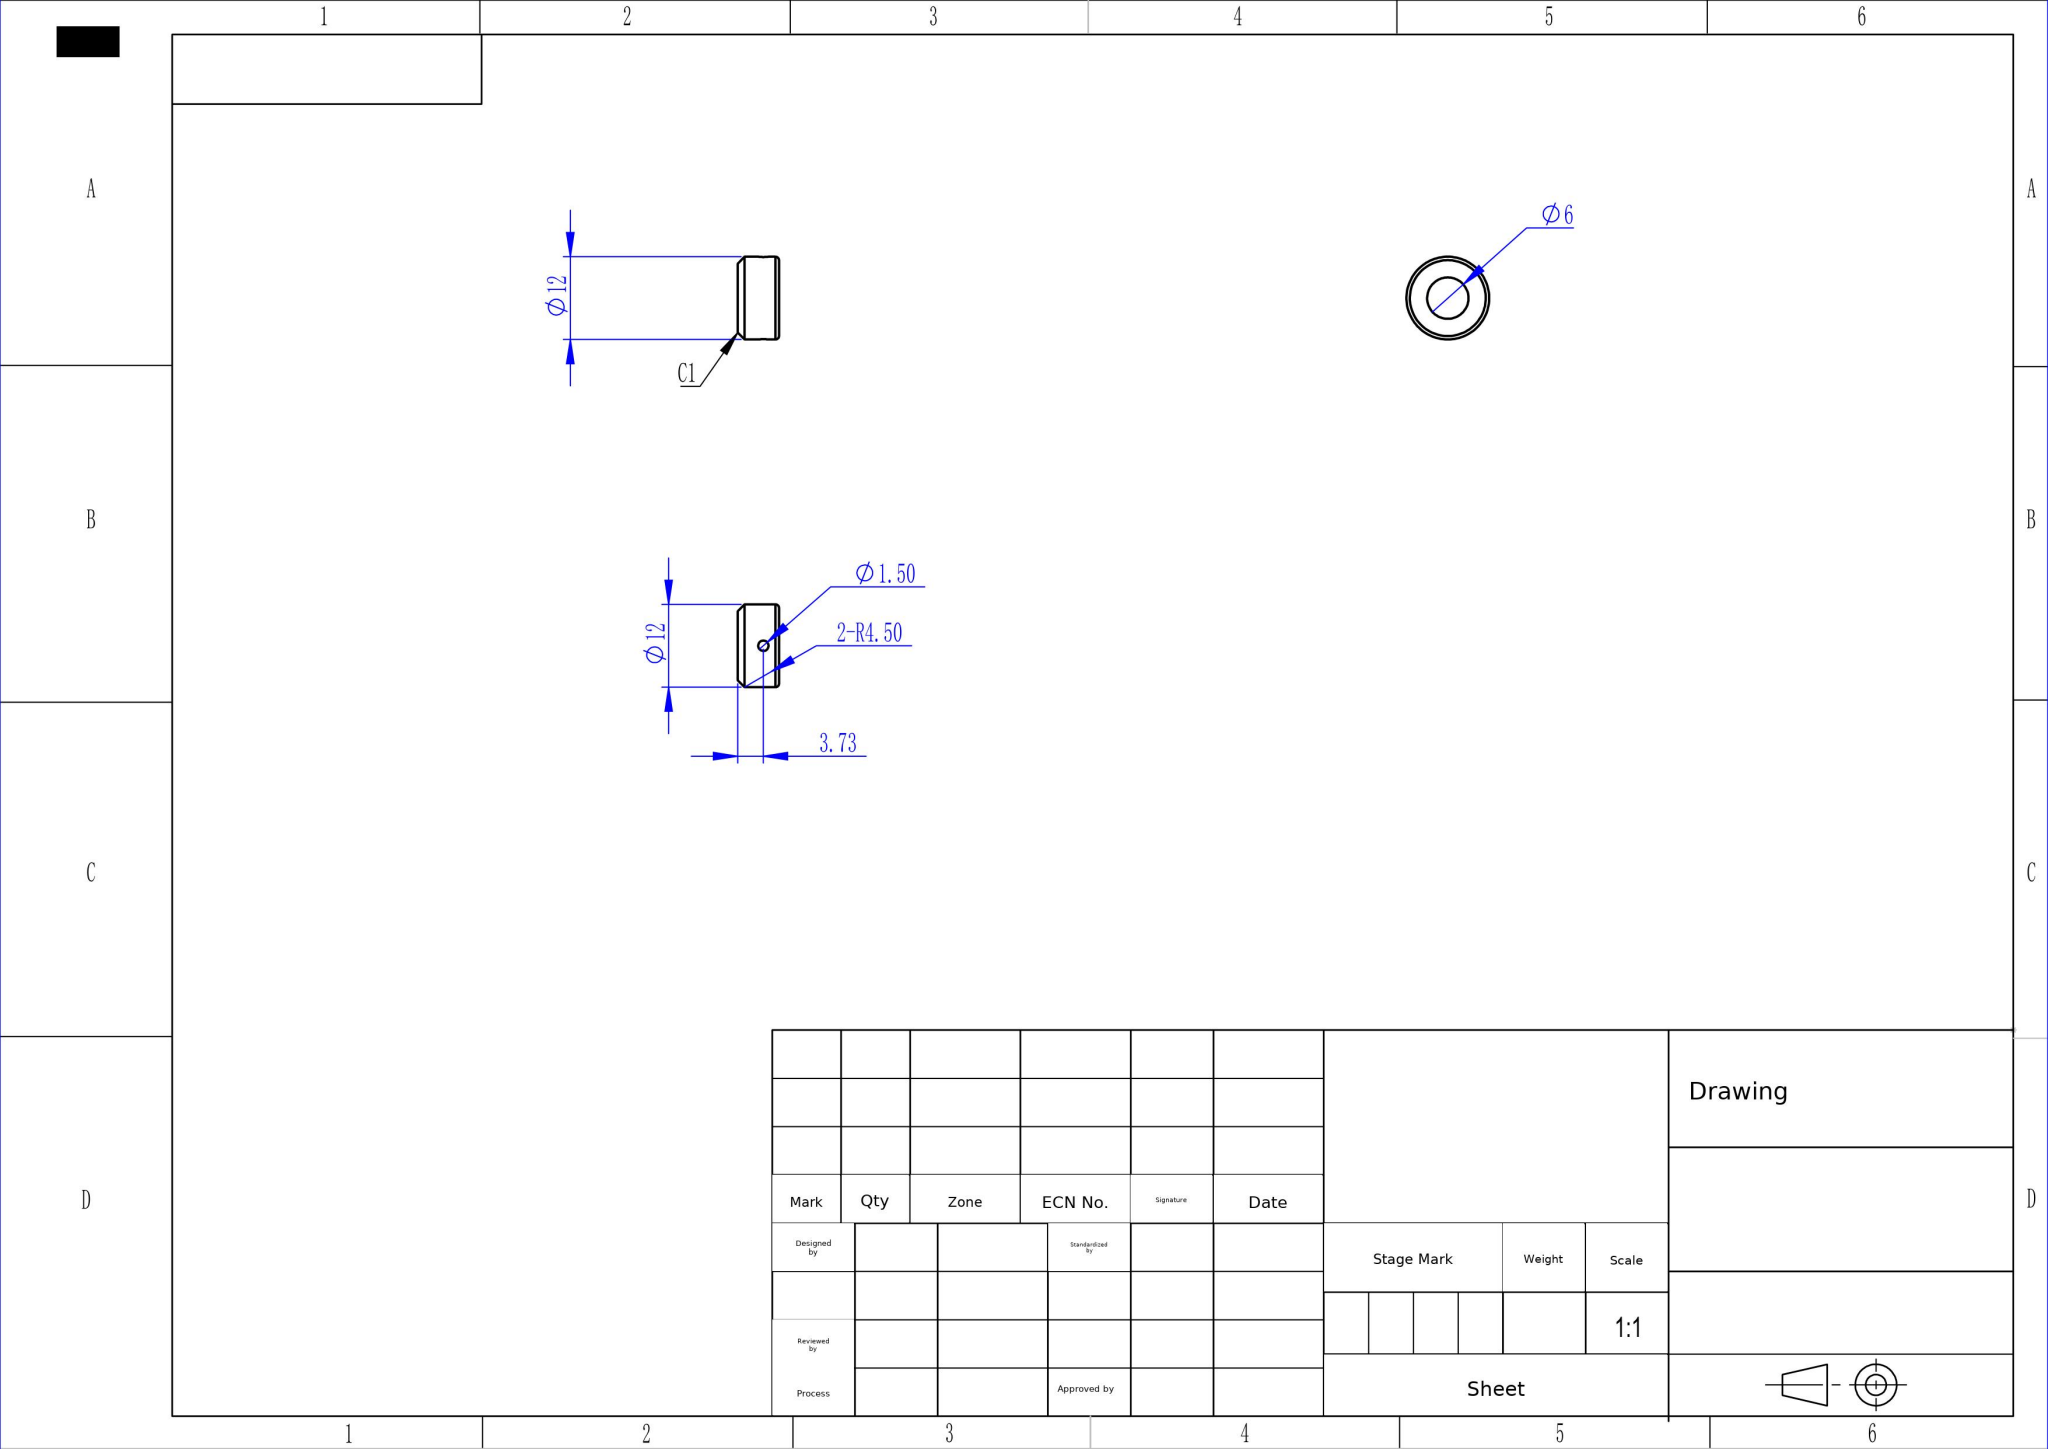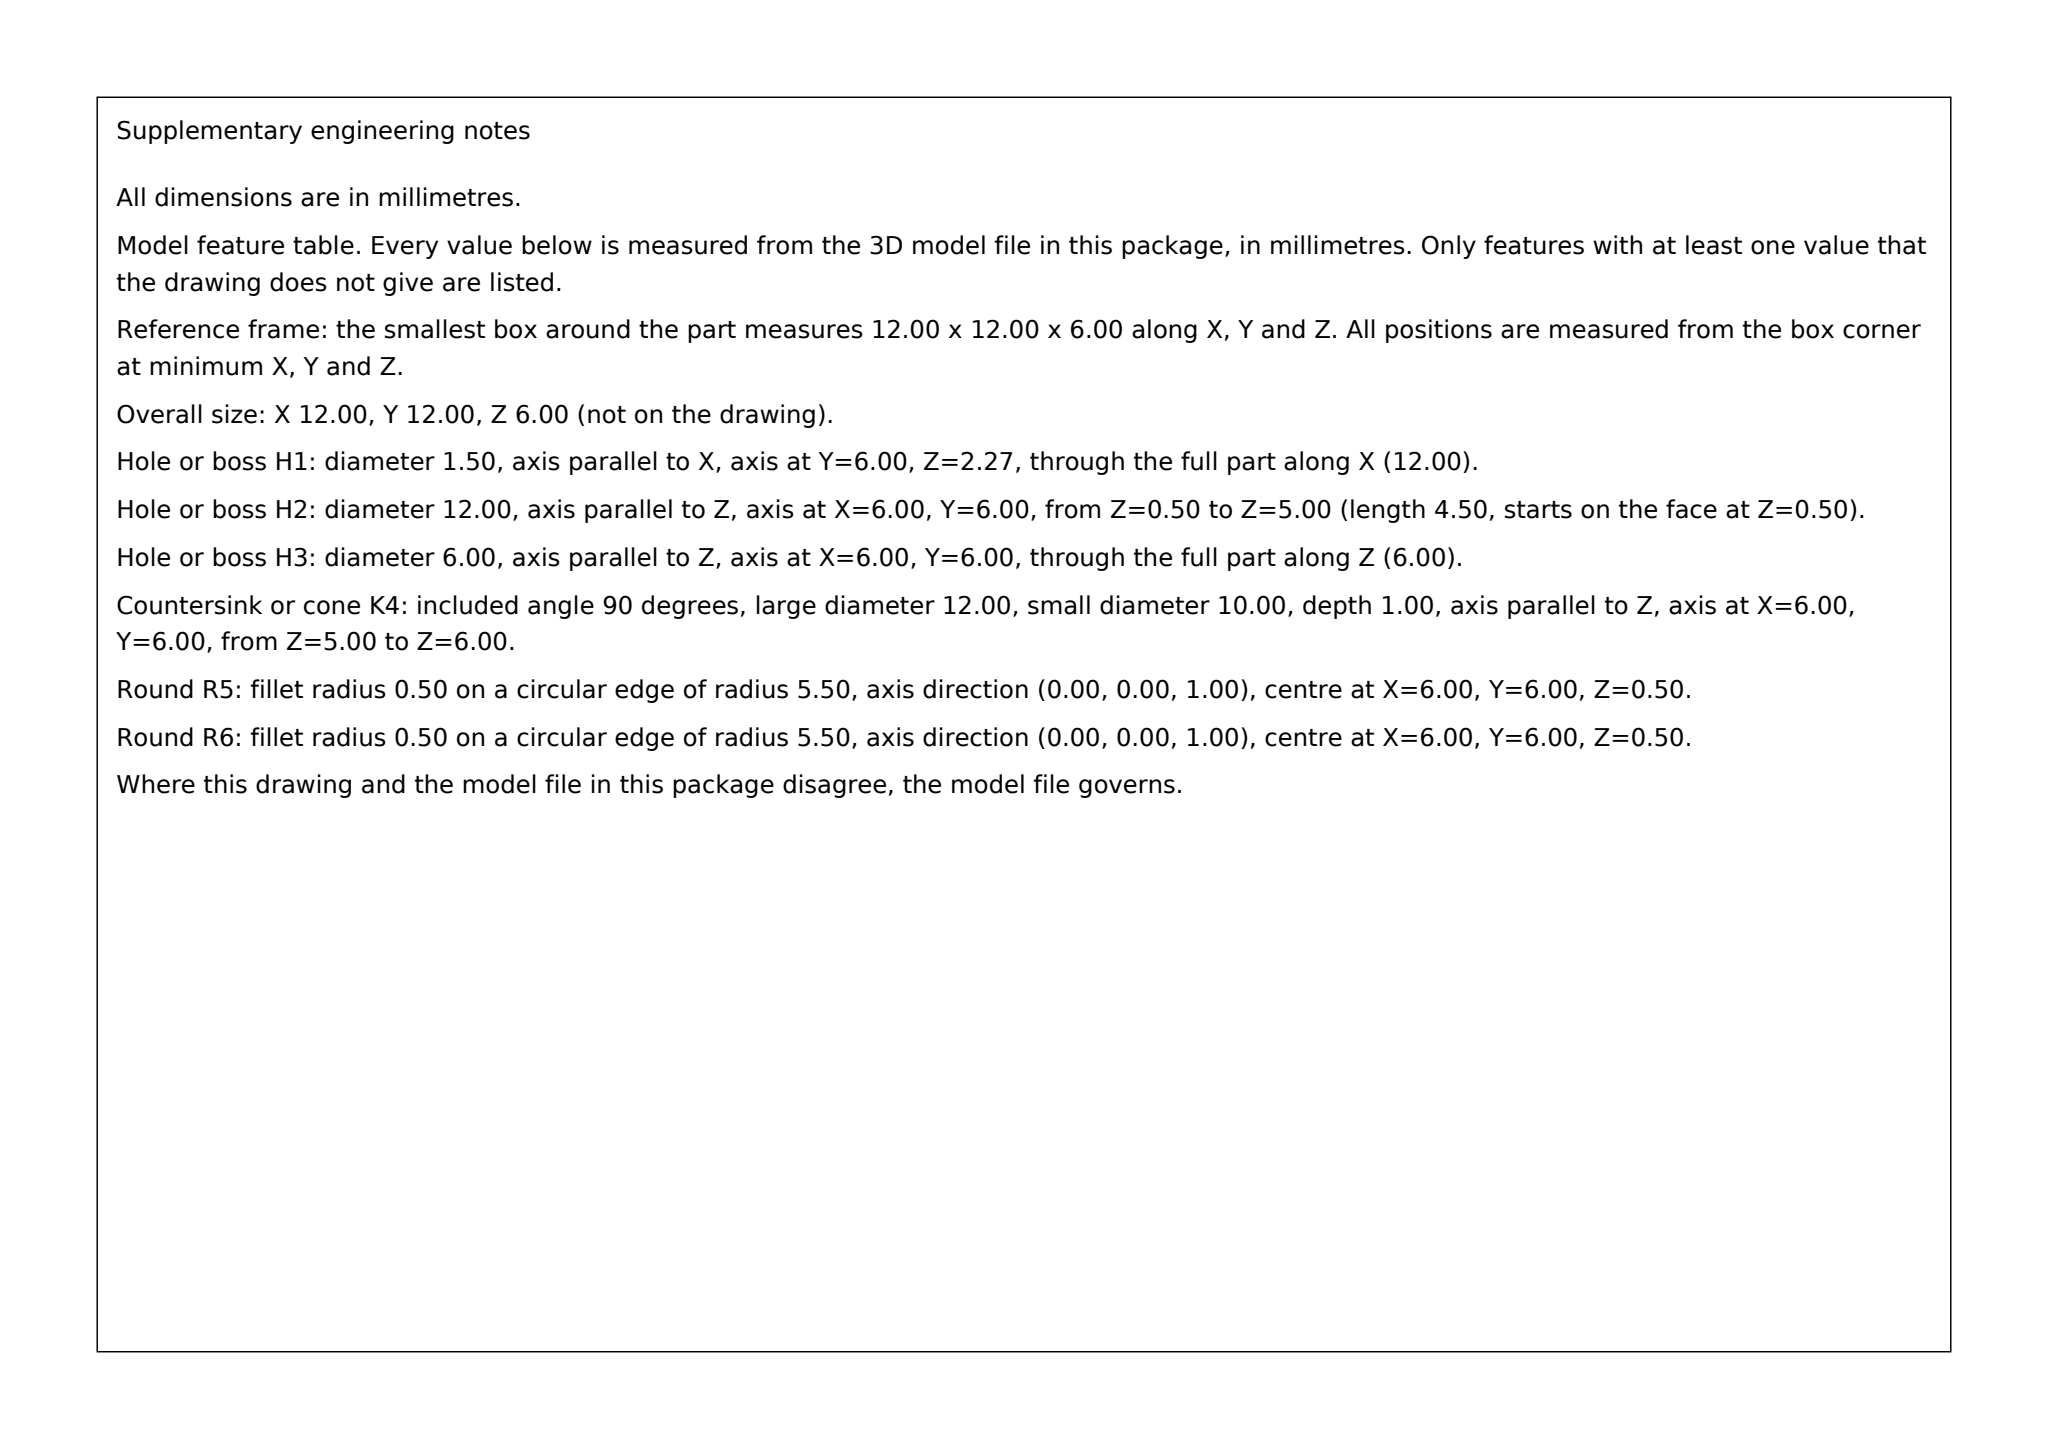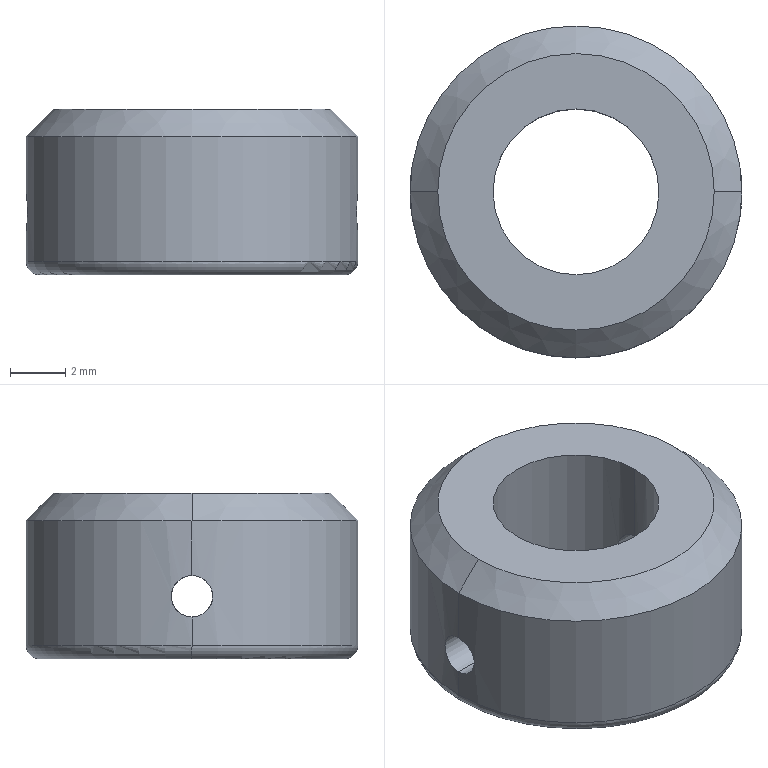Part | SolidWorks | mm | 1 solid | 14 faces | box 12 x 12 x 6 mm | volume 479 mm3 | cylinder 8 | cone 2 | torus 2 | plane 2 | commonest cylinder face diameters 1.5 x4 6 x2 12 x2
build123d program:
from build123d import *

# Parameters (mm, degrees)
SKETCH1_R               = 6
SKETCH1_R_2             = 3
BOSS_EXTRUDE1_DEPTH     = 6
FILLET1_R               = 0.5
CHAMFER1_SIZE           = 1
CUT_EXTRUDE1_DEPTH      = 11.392
CUT_EXTRUDE1_DEPTH_BACK = 11.392
SKETCH2_R               = 0.75


with BuildPart() as part:
    # Sketch1 → Boss-Extrude1 (new body)
    with BuildSketch(Plane.XY):
        Circle(SKETCH1_R)
        Circle(SKETCH1_R_2, mode=Mode.SUBTRACT)
    extrude(amount=BOSS_EXTRUDE1_DEPTH)

    # Fillet1
    fillet1_edges = [part.edges().sort_by_distance(p)[0] for p in [
        (-6, 0, 0),
    ]]
    fillet(fillet1_edges, radius=FILLET1_R)

    # Chamfer1
    chamfer1_edges = [part.edges().sort_by_distance(p)[0] for p in [
        (-6, 0, 6),
    ]]
    chamfer(chamfer1_edges, length=CHAMFER1_SIZE)

    # Sketch2 → Cut-Extrude1 (cut, two sides: drawn at the far end of the back side and taken through both)
    with BuildSketch(Plane(origin=(0, 0, 0), x_dir=(0, 0, -1), z_dir=(1, 0, 0)).offset(-CUT_EXTRUDE1_DEPTH_BACK)):
        with Locations((-2.267, 0)):
            Circle(SKETCH2_R)
    extrude(amount=CUT_EXTRUDE1_DEPTH + CUT_EXTRUDE1_DEPTH_BACK, mode=Mode.SUBTRACT)


solid = part.part
STEP:
#1=CARTESIAN_POINT('',(-6.,0.,3.017));
#2=VERTEX_POINT('',#1);
#3=CARTESIAN_POINT('',(-6.,0.,1.517));
#4=VERTEX_POINT('',#3);
#5=CARTESIAN_POINT('',(-6.,0.,3.017));
#6=CARTESIAN_POINT('',(-6.,-0.1958,3.017));
#7=CARTESIAN_POINT('',(-5.989,-0.3916,2.936));
#8=CARTESIAN_POINT('',(-5.97,-0.5992,2.729));
#9=CARTESIAN_POINT('',(-5.964,-0.6549,2.646));
#10=CARTESIAN_POINT('',(-5.956,-0.7303,2.464));
#11=CARTESIAN_POINT('',(-5.953,-0.7499,2.367));
#12=CARTESIAN_POINT('',(-5.953,-0.7501,2.169));
#13=CARTESIAN_POINT('',(-5.955,-0.7306,2.071));
#14=CARTESIAN_POINT('',(-5.964,-0.6554,1.89));
#15=CARTESIAN_POINT('',(-5.97,-0.5997,1.806));
#16=CARTESIAN_POINT('',(-5.989,-0.3926,1.599));
#17=CARTESIAN_POINT('',(-6.,-0.1984,1.517));
#18=CARTESIAN_POINT('',(-6.,0.,1.517));
#19=B_SPLINE_CURVE_WITH_KNOTS('',3,(#5,#6,#7,#8,#9,#10,#11,#12,#13,#14,#15,#16,#17,#18),.UNSPECIFIED.,.F.,.F.,(4,2,2,2,2,2,4),(0.002347,0.002934,0.003227,0.00352,0.003814,0.004107,0.004694),.UNSPECIFIED.);
#20=EDGE_CURVE('',#2,#4,#19,.T.);
#21=ORIENTED_EDGE('',*,*,#20,.F.);
#22=CARTESIAN_POINT('',(-3.,0.,3.017));
#23=VERTEX_POINT('',#22);
#24=CARTESIAN_POINT('',(-6.,0.,3.017));
#25=DIRECTION('',(1.,0.,0.));
#26=VECTOR('',#25,1000.);
#27=LINE('',#24,#26);
#28=EDGE_CURVE('',#2,#23,#27,.T.);
#29=ORIENTED_EDGE('',*,*,#28,.T.);
#30=CARTESIAN_POINT('',(-3.,0.,1.517));
#31=VERTEX_POINT('',#30);
#32=CARTESIAN_POINT('',(-3.,0.,3.017));
#33=CARTESIAN_POINT('',(-3.,-0.09953,3.017));
#34=CARTESIAN_POINT('',(-2.995,-0.1972,2.998));
#35=CARTESIAN_POINT('',(-2.977,-0.3787,2.922));
#36=CARTESIAN_POINT('',(-2.965,-0.4616,2.866));
#37=CARTESIAN_POINT('',(-2.94,-0.5994,2.729));
#38=CARTESIAN_POINT('',(-2.928,-0.6552,2.645));
#39=CARTESIAN_POINT('',(-2.91,-0.7301,2.465));
#40=CARTESIAN_POINT('',(-2.905,-0.75,2.366));
#41=CARTESIAN_POINT('',(-2.905,-0.75,2.169));
#42=CARTESIAN_POINT('',(-2.91,-0.7305,2.071));
#43=CARTESIAN_POINT('',(-2.928,-0.6549,1.889));
#44=CARTESIAN_POINT('',(-2.94,-0.5997,1.806));
#45=CARTESIAN_POINT('',(-2.965,-0.4607,1.667));
#46=CARTESIAN_POINT('',(-2.977,-0.3781,1.612));
#47=CARTESIAN_POINT('',(-2.995,-0.197,1.537));
#48=CARTESIAN_POINT('',(-3.,-0.09813,1.517));
#49=CARTESIAN_POINT('',(-3.,0.,1.517));
#50=B_SPLINE_CURVE_WITH_KNOTS('',3,(#32,#33,#34,#35,#36,#37,#38,#39,#40,#41,#42,#43,#44,#45,#46,#47,#48,#49),.UNSPECIFIED.,.F.,.F.,(4,2,2,2,2,2,2,2,4),(0.,0.0002943,0.0005886,0.0008828,0.001177,0.001471,0.001766,0.00206,0.002354),.UNSPECIFIED.);
#51=EDGE_CURVE('',#23,#31,#50,.T.);
#52=ORIENTED_EDGE('',*,*,#51,.T.);
#53=CARTESIAN_POINT('',(-6.,0.,1.517));
#54=DIRECTION('',(1.,0.,0.));
#55=VECTOR('',#54,1000.);
#56=LINE('',#53,#55);
#57=EDGE_CURVE('',#4,#31,#56,.T.);
#58=ORIENTED_EDGE('',*,*,#57,.F.);
#59=EDGE_LOOP('',(#21,#29,#52,#58));
#60=FACE_OUTER_BOUND('',#59,.T.);
#61=CARTESIAN_POINT('',(-6.,0.,2.267));
#62=DIRECTION('',(1.,0.,0.));
#63=DIRECTION('',(0.,0.,-1.));
#64=AXIS2_PLACEMENT_3D('',#61,#62,#63);
#65=CYLINDRICAL_SURFACE('',#64,0.75);
#66=ADVANCED_FACE('',(#60),#65,.F.);
#67=CARTESIAN_POINT('',(3.,-0.,1.517));
#68=VERTEX_POINT('',#67);
#69=CARTESIAN_POINT('',(3.,0.,3.017));
#70=VERTEX_POINT('',#69);
#71=CARTESIAN_POINT('',(3.,-0.,1.517));
#72=CARTESIAN_POINT('',(3.,-0.09953,1.517));
#73=CARTESIAN_POINT('',(2.995,-0.1972,1.537));
#74=CARTESIAN_POINT('',(2.977,-0.3787,1.612));
#75=CARTESIAN_POINT('',(2.965,-0.4616,1.668));
#76=CARTESIAN_POINT('',(2.94,-0.5994,1.806));
#77=CARTESIAN_POINT('',(2.928,-0.6552,1.889));
#78=CARTESIAN_POINT('',(2.91,-0.7301,2.07));
#79=CARTESIAN_POINT('',(2.905,-0.75,2.169));
#80=CARTESIAN_POINT('',(2.905,-0.75,2.365));
#81=CARTESIAN_POINT('',(2.91,-0.7305,2.464));
#82=CARTESIAN_POINT('',(2.928,-0.6549,2.646));
#83=CARTESIAN_POINT('',(2.94,-0.5997,2.728));
#84=CARTESIAN_POINT('',(2.965,-0.4607,2.867));
#85=CARTESIAN_POINT('',(2.977,-0.3781,2.922));
#86=CARTESIAN_POINT('',(2.995,-0.197,2.998));
#87=CARTESIAN_POINT('',(3.,-0.09813,3.017));
#88=CARTESIAN_POINT('',(3.,0.,3.017));
#89=B_SPLINE_CURVE_WITH_KNOTS('',3,(#71,#72,#73,#74,#75,#76,#77,#78,#79,#80,#81,#82,#83,#84,#85,#86,#87,#88),.UNSPECIFIED.,.F.,.F.,(4,2,2,2,2,2,2,2,4),(0.,0.0002943,0.0005886,0.0008828,0.001177,0.001471,0.001766,0.00206,0.002354),.UNSPECIFIED.);
#90=EDGE_CURVE('',#68,#70,#89,.T.);
#91=ORIENTED_EDGE('',*,*,#90,.T.);
#92=CARTESIAN_POINT('',(6.,-0.,3.017));
#93=VERTEX_POINT('',#92);
#94=CARTESIAN_POINT('',(-6.,0.,3.017));
#95=DIRECTION('',(1.,0.,0.));
#96=VECTOR('',#95,1000.);
#97=LINE('',#94,#96);
#98=EDGE_CURVE('',#70,#93,#97,.T.);
#99=ORIENTED_EDGE('',*,*,#98,.T.);
#100=CARTESIAN_POINT('',(6.,0.,1.517));
#101=VERTEX_POINT('',#100);
#102=CARTESIAN_POINT('',(6.,0.,1.517));
#103=CARTESIAN_POINT('',(6.,-0.09921,1.517));
#104=CARTESIAN_POINT('',(5.997,-0.1966,1.537));
#105=CARTESIAN_POINT('',(5.989,-0.3782,1.612));
#106=CARTESIAN_POINT('',(5.983,-0.4613,1.668));
#107=CARTESIAN_POINT('',(5.964,-0.6687,1.875));
#108=CARTESIAN_POINT('',(5.953,-0.7499,2.071));
#109=CARTESIAN_POINT('',(5.953,-0.75,2.365));
#110=CARTESIAN_POINT('',(5.955,-0.7306,2.463));
#111=CARTESIAN_POINT('',(5.964,-0.6553,2.645));
#112=CARTESIAN_POINT('',(5.97,-0.6004,2.728));
#113=CARTESIAN_POINT('',(5.983,-0.4604,2.868));
#114=CARTESIAN_POINT('',(5.989,-0.3779,2.923));
#115=CARTESIAN_POINT('',(5.997,-0.1963,2.998));
#116=CARTESIAN_POINT('',(6.,-0.09795,3.017));
#117=CARTESIAN_POINT('',(6.,-0.,3.017));
#118=B_SPLINE_CURVE_WITH_KNOTS('',3,(#102,#103,#104,#105,#106,#107,#108,#109,#110,#111,#112,#113,#114,#115,#116,#117),.UNSPECIFIED.,.F.,.F.,(4,2,2,2,2,2,2,4),(0.,0.0002934,0.0005868,0.001174,0.001467,0.00176,0.002054,0.002347),.UNSPECIFIED.);
#119=EDGE_CURVE('',#101,#93,#118,.T.);
#120=ORIENTED_EDGE('',*,*,#119,.F.);
#121=CARTESIAN_POINT('',(-6.,0.,1.517));
#122=DIRECTION('',(1.,0.,0.));
#123=VECTOR('',#122,1000.);
#124=LINE('',#121,#123);
#125=EDGE_CURVE('',#68,#101,#124,.T.);
#126=ORIENTED_EDGE('',*,*,#125,.F.);
#127=EDGE_LOOP('',(#91,#99,#120,#126));
#128=FACE_OUTER_BOUND('',#127,.T.);
#129=CARTESIAN_POINT('',(-6.,0.,2.267));
#130=DIRECTION('',(1.,0.,0.));
#131=DIRECTION('',(0.,0.,-1.));
#132=AXIS2_PLACEMENT_3D('',#129,#130,#131);
#133=CYLINDRICAL_SURFACE('',#132,0.75);
#134=ADVANCED_FACE('',(#128),#133,.F.);
#135=CARTESIAN_POINT('',(5.,0.,6.));
#136=VERTEX_POINT('',#135);
#137=CARTESIAN_POINT('',(-5.,0.,6.));
#138=VERTEX_POINT('',#137);
#139=CARTESIAN_POINT('',(0.,0.,6.));
#140=DIRECTION('',(0.,0.,1.));
#141=DIRECTION('',(1.,0.,0.));
#142=AXIS2_PLACEMENT_3D('',#139,#140,#141);
#143=CIRCLE('',#142,5.);
#144=EDGE_CURVE('',#136,#138,#143,.T.);
#145=ORIENTED_EDGE('',*,*,#144,.F.);
#146=CARTESIAN_POINT('',(6.,0.,5.));
#147=VERTEX_POINT('',#146);
#148=CARTESIAN_POINT('',(5.,0.,6.));
#149=DIRECTION('',(0.7071,0.,-0.7071));
#150=VECTOR('',#149,1000.);
#151=LINE('',#148,#150);
#152=EDGE_CURVE('',#136,#147,#151,.T.);
#153=ORIENTED_EDGE('',*,*,#152,.T.);
#154=CARTESIAN_POINT('',(-6.,0.,5.));
#155=VERTEX_POINT('',#154);
#156=CARTESIAN_POINT('',(0.,0.,5.));
#157=DIRECTION('',(0.,0.,-1.));
#158=DIRECTION('',(1.,0.,0.));
#159=AXIS2_PLACEMENT_3D('',#156,#157,#158);
#160=CIRCLE('',#159,6.);
#161=EDGE_CURVE('',#155,#147,#160,.T.);
#162=ORIENTED_EDGE('',*,*,#161,.F.);
#163=CARTESIAN_POINT('',(-5.,0.,6.));
#164=DIRECTION('',(-0.7071,0.,-0.7071));
#165=VECTOR('',#164,1000.);
#166=LINE('',#163,#165);
#167=EDGE_CURVE('',#138,#155,#166,.T.);
#168=ORIENTED_EDGE('',*,*,#167,.F.);
#169=EDGE_LOOP('',(#145,#153,#162,#168));
#170=FACE_OUTER_BOUND('',#169,.T.);
#171=CARTESIAN_POINT('',(0.,0.,6.));
#172=DIRECTION('',(0.,0.,-1.));
#173=DIRECTION('',(-1.,0.,0.));
#174=AXIS2_PLACEMENT_3D('',#171,#172,#173);
#175=CONICAL_SURFACE('',#174,5.,0.7854);
#176=ADVANCED_FACE('',(#170),#175,.T.);
#177=CARTESIAN_POINT('',(-5.5,0.,0.));
#178=VERTEX_POINT('',#177);
#179=CARTESIAN_POINT('',(5.5,0.,0.));
#180=VERTEX_POINT('',#179);
#181=CARTESIAN_POINT('',(0.,0.,0.));
#182=DIRECTION('',(0.,0.,-1.));
#183=DIRECTION('',(1.,0.,0.));
#184=AXIS2_PLACEMENT_3D('',#181,#182,#183);
#185=CIRCLE('',#184,5.5);
#186=EDGE_CURVE('',#178,#180,#185,.T.);
#187=ORIENTED_EDGE('',*,*,#186,.F.);
#188=CARTESIAN_POINT('',(-6.,0.,0.5));
#189=VERTEX_POINT('',#188);
#190=CARTESIAN_POINT('',(-5.5,0.,0.5));
#191=DIRECTION('',(0.,1.,0.));
#192=DIRECTION('',(-1.,0.,0.));
#193=AXIS2_PLACEMENT_3D('',#190,#191,#192);
#194=CIRCLE('',#193,0.5);
#195=EDGE_CURVE('',#178,#189,#194,.T.);
#196=ORIENTED_EDGE('',*,*,#195,.T.);
#197=CARTESIAN_POINT('',(6.,0.,0.5));
#198=VERTEX_POINT('',#197);
#199=CARTESIAN_POINT('',(0.,0.,0.5));
#200=DIRECTION('',(0.,0.,1.));
#201=DIRECTION('',(1.,0.,0.));
#202=AXIS2_PLACEMENT_3D('',#199,#200,#201);
#203=CIRCLE('',#202,6.);
#204=EDGE_CURVE('',#198,#189,#203,.T.);
#205=ORIENTED_EDGE('',*,*,#204,.F.);
#206=CARTESIAN_POINT('',(5.5,0.,0.5));
#207=DIRECTION('',(0.,-1.,0.));
#208=DIRECTION('',(0.,0.,-1.));
#209=AXIS2_PLACEMENT_3D('',#206,#207,#208);
#210=CIRCLE('',#209,0.5);
#211=EDGE_CURVE('',#180,#198,#210,.T.);
#212=ORIENTED_EDGE('',*,*,#211,.F.);
#213=EDGE_LOOP('',(#187,#196,#205,#212));
#214=FACE_OUTER_BOUND('',#213,.T.);
#215=CARTESIAN_POINT('',(0.,0.,0.5));
#216=DIRECTION('',(0.,0.,1.));
#217=DIRECTION('',(1.,0.,0.));
#218=AXIS2_PLACEMENT_3D('',#215,#216,#217);
#219=TOROIDAL_SURFACE('',#218,5.5,0.5);
#220=ADVANCED_FACE('',(#214),#219,.T.);
#221=CARTESIAN_POINT('',(-3.,0.,6.));
#222=VERTEX_POINT('',#221);
#223=CARTESIAN_POINT('',(3.,0.,6.));
#224=VERTEX_POINT('',#223);
#225=CARTESIAN_POINT('',(0.,0.,6.));
#226=DIRECTION('',(0.,0.,1.));
#227=DIRECTION('',(1.,0.,0.));
#228=AXIS2_PLACEMENT_3D('',#225,#226,#227);
#229=CIRCLE('',#228,3.);
#230=EDGE_CURVE('',#222,#224,#229,.T.);
#231=ORIENTED_EDGE('',*,*,#230,.T.);
#232=CARTESIAN_POINT('',(3.,0.,6.));
#233=DIRECTION('',(0.,0.,-1.));
#234=VECTOR('',#233,1000.);
#235=LINE('',#232,#234);
#236=EDGE_CURVE('',#224,#70,#235,.T.);
#237=ORIENTED_EDGE('',*,*,#236,.T.);
#238=ORIENTED_EDGE('',*,*,#90,.F.);
#239=CARTESIAN_POINT('',(3.,0.,0.));
#240=VERTEX_POINT('',#239);
#241=CARTESIAN_POINT('',(3.,0.,6.));
#242=DIRECTION('',(0.,0.,-1.));
#243=VECTOR('',#242,1000.);
#244=LINE('',#241,#243);
#245=EDGE_CURVE('',#68,#240,#244,.T.);
#246=ORIENTED_EDGE('',*,*,#245,.T.);
#247=CARTESIAN_POINT('',(-3.,0.,0.));
#248=VERTEX_POINT('',#247);
#249=CARTESIAN_POINT('',(0.,0.,0.));
#250=DIRECTION('',(0.,0.,1.));
#251=DIRECTION('',(1.,0.,0.));
#252=AXIS2_PLACEMENT_3D('',#249,#250,#251);
#253=CIRCLE('',#252,3.);
#254=EDGE_CURVE('',#248,#240,#253,.T.);
#255=ORIENTED_EDGE('',*,*,#254,.F.);
#256=CARTESIAN_POINT('',(-3.,0.,6.));
#257=DIRECTION('',(0.,0.,-1.));
#258=VECTOR('',#257,1000.);
#259=LINE('',#256,#258);
#260=EDGE_CURVE('',#31,#248,#259,.T.);
#261=ORIENTED_EDGE('',*,*,#260,.F.);
#262=ORIENTED_EDGE('',*,*,#51,.F.);
#263=CARTESIAN_POINT('',(-3.,0.,6.));
#264=DIRECTION('',(0.,0.,-1.));
#265=VECTOR('',#264,1000.);
#266=LINE('',#263,#265);
#267=EDGE_CURVE('',#222,#23,#266,.T.);
#268=ORIENTED_EDGE('',*,*,#267,.F.);
#269=EDGE_LOOP('',(#231,#237,#238,#246,#255,#261,#262,#268));
#270=FACE_OUTER_BOUND('',#269,.T.);
#271=CARTESIAN_POINT('',(0.,0.,6.));
#272=DIRECTION('',(0.,0.,-1.));
#273=DIRECTION('',(-1.,0.,0.));
#274=AXIS2_PLACEMENT_3D('',#271,#272,#273);
#275=CYLINDRICAL_SURFACE('',#274,3.);
#276=ADVANCED_FACE('',(#270),#275,.F.);
#277=ORIENTED_EDGE('',*,*,#161,.T.);
#278=CARTESIAN_POINT('',(6.,0.,6.));
#279=DIRECTION('',(0.,0.,-1.));
#280=VECTOR('',#279,1000.);
#281=LINE('',#278,#280);
#282=EDGE_CURVE('',#147,#93,#281,.T.);
#283=ORIENTED_EDGE('',*,*,#282,.T.);
#284=CARTESIAN_POINT('',(6.,-0.,3.017));
#285=CARTESIAN_POINT('',(6.,0.1958,3.017));
#286=CARTESIAN_POINT('',(5.989,0.3916,2.936));
#287=CARTESIAN_POINT('',(5.97,0.5992,2.729));
#288=CARTESIAN_POINT('',(5.964,0.6549,2.646));
#289=CARTESIAN_POINT('',(5.956,0.7303,2.464));
#290=CARTESIAN_POINT('',(5.953,0.7499,2.367));
#291=CARTESIAN_POINT('',(5.953,0.7501,2.169));
#292=CARTESIAN_POINT('',(5.955,0.7306,2.071));
#293=CARTESIAN_POINT('',(5.964,0.6554,1.89));
#294=CARTESIAN_POINT('',(5.97,0.5997,1.806));
#295=CARTESIAN_POINT('',(5.989,0.3926,1.599));
#296=CARTESIAN_POINT('',(6.,0.1984,1.517));
#297=CARTESIAN_POINT('',(6.,0.,1.517));
#298=B_SPLINE_CURVE_WITH_KNOTS('',3,(#284,#285,#286,#287,#288,#289,#290,#291,#292,#293,#294,#295,#296,#297),.UNSPECIFIED.,.F.,.F.,(4,2,2,2,2,2,4),(0.002347,0.002934,0.003227,0.00352,0.003814,0.004107,0.004694),.UNSPECIFIED.);
#299=EDGE_CURVE('',#93,#101,#298,.T.);
#300=ORIENTED_EDGE('',*,*,#299,.T.);
#301=CARTESIAN_POINT('',(6.,0.,6.));
#302=DIRECTION('',(0.,0.,-1.));
#303=VECTOR('',#302,1000.);
#304=LINE('',#301,#303);
#305=EDGE_CURVE('',#101,#198,#304,.T.);
#306=ORIENTED_EDGE('',*,*,#305,.T.);
#307=ORIENTED_EDGE('',*,*,#204,.T.);
#308=CARTESIAN_POINT('',(-6.,0.,6.));
#309=DIRECTION('',(0.,0.,-1.));
#310=VECTOR('',#309,1000.);
#311=LINE('',#308,#310);
#312=EDGE_CURVE('',#4,#189,#311,.T.);
#313=ORIENTED_EDGE('',*,*,#312,.F.);
#314=CARTESIAN_POINT('',(-6.,0.,1.517));
#315=CARTESIAN_POINT('',(-6.,0.09921,1.517));
#316=CARTESIAN_POINT('',(-5.997,0.1966,1.537));
#317=CARTESIAN_POINT('',(-5.989,0.3782,1.612));
#318=CARTESIAN_POINT('',(-5.983,0.4613,1.668));
#319=CARTESIAN_POINT('',(-5.964,0.6687,1.875));
#320=CARTESIAN_POINT('',(-5.953,0.7499,2.071));
#321=CARTESIAN_POINT('',(-5.953,0.75,2.365));
#322=CARTESIAN_POINT('',(-5.955,0.7306,2.463));
#323=CARTESIAN_POINT('',(-5.964,0.6553,2.645));
#324=CARTESIAN_POINT('',(-5.97,0.6004,2.728));
#325=CARTESIAN_POINT('',(-5.983,0.4604,2.868));
#326=CARTESIAN_POINT('',(-5.989,0.3779,2.923));
#327=CARTESIAN_POINT('',(-5.997,0.1963,2.998));
#328=CARTESIAN_POINT('',(-6.,0.09795,3.017));
#329=CARTESIAN_POINT('',(-6.,0.,3.017));
#330=B_SPLINE_CURVE_WITH_KNOTS('',3,(#314,#315,#316,#317,#318,#319,#320,#321,#322,#323,#324,#325,#326,#327,#328,#329),.UNSPECIFIED.,.F.,.F.,(4,2,2,2,2,2,2,4),(0.,0.0002934,0.0005868,0.001174,0.001467,0.00176,0.002054,0.002347),.UNSPECIFIED.);
#331=EDGE_CURVE('',#4,#2,#330,.T.);
#332=ORIENTED_EDGE('',*,*,#331,.T.);
#333=CARTESIAN_POINT('',(-6.,0.,6.));
#334=DIRECTION('',(0.,0.,-1.));
#335=VECTOR('',#334,1000.);
#336=LINE('',#333,#335);
#337=EDGE_CURVE('',#155,#2,#336,.T.);
#338=ORIENTED_EDGE('',*,*,#337,.F.);
#339=EDGE_LOOP('',(#277,#283,#300,#306,#307,#313,#332,#338));
#340=FACE_OUTER_BOUND('',#339,.T.);
#341=CARTESIAN_POINT('',(0.,0.,6.));
#342=DIRECTION('',(0.,0.,-1.));
#343=DIRECTION('',(-1.,0.,0.));
#344=AXIS2_PLACEMENT_3D('',#341,#342,#343);
#345=CYLINDRICAL_SURFACE('',#344,6.);
#346=ADVANCED_FACE('',(#340),#345,.T.);
#347=CARTESIAN_POINT('',(0.,0.,6.));
#348=DIRECTION('',(0.,0.,1.));
#349=DIRECTION('',(1.,0.,0.));
#350=AXIS2_PLACEMENT_3D('',#347,#348,#349);
#351=CIRCLE('',#350,5.);
#352=EDGE_CURVE('',#138,#136,#351,.T.);
#353=ORIENTED_EDGE('',*,*,#352,.T.);
#354=ORIENTED_EDGE('',*,*,#144,.T.);
#355=EDGE_LOOP('',(#353,#354));
#356=FACE_OUTER_BOUND('',#355,.T.);
#357=ORIENTED_EDGE('',*,*,#230,.F.);
#358=CARTESIAN_POINT('',(0.,0.,6.));
#359=DIRECTION('',(0.,0.,1.));
#360=DIRECTION('',(1.,0.,0.));
#361=AXIS2_PLACEMENT_3D('',#358,#359,#360);
#362=CIRCLE('',#361,3.);
#363=EDGE_CURVE('',#224,#222,#362,.T.);
#364=ORIENTED_EDGE('',*,*,#363,.F.);
#365=EDGE_LOOP('',(#357,#364));
#366=FACE_BOUND('',#365,.T.);
#367=CARTESIAN_POINT('',(0.,0.,6.));
#368=DIRECTION('',(0.,0.,1.));
#369=DIRECTION('',(1.,0.,0.));
#370=AXIS2_PLACEMENT_3D('',#367,#368,#369);
#371=PLANE('',#370);
#372=ADVANCED_FACE('',(#356,#366),#371,.T.);
#373=CARTESIAN_POINT('',(0.,0.,0.));
#374=DIRECTION('',(0.,0.,-1.));
#375=DIRECTION('',(1.,0.,0.));
#376=AXIS2_PLACEMENT_3D('',#373,#374,#375);
#377=CIRCLE('',#376,5.5);
#378=EDGE_CURVE('',#180,#178,#377,.T.);
#379=ORIENTED_EDGE('',*,*,#378,.T.);
#380=ORIENTED_EDGE('',*,*,#186,.T.);
#381=EDGE_LOOP('',(#379,#380));
#382=FACE_OUTER_BOUND('',#381,.T.);
#383=ORIENTED_EDGE('',*,*,#254,.T.);
#384=CARTESIAN_POINT('',(0.,0.,0.));
#385=DIRECTION('',(0.,0.,1.));
#386=DIRECTION('',(1.,0.,0.));
#387=AXIS2_PLACEMENT_3D('',#384,#385,#386);
#388=CIRCLE('',#387,3.);
#389=EDGE_CURVE('',#240,#248,#388,.T.);
#390=ORIENTED_EDGE('',*,*,#389,.T.);
#391=EDGE_LOOP('',(#383,#390));
#392=FACE_BOUND('',#391,.T.);
#393=CARTESIAN_POINT('',(0.,0.,0.));
#394=DIRECTION('',(0.,0.,1.));
#395=DIRECTION('',(1.,0.,0.));
#396=AXIS2_PLACEMENT_3D('',#393,#394,#395);
#397=PLANE('',#396);
#398=ADVANCED_FACE('',(#382,#392),#397,.F.);
#399=ORIENTED_EDGE('',*,*,#282,.F.);
#400=CARTESIAN_POINT('',(0.,0.,5.));
#401=DIRECTION('',(0.,0.,-1.));
#402=DIRECTION('',(1.,0.,0.));
#403=AXIS2_PLACEMENT_3D('',#400,#401,#402);
#404=CIRCLE('',#403,6.);
#405=EDGE_CURVE('',#147,#155,#404,.T.);
#406=ORIENTED_EDGE('',*,*,#405,.T.);
#407=ORIENTED_EDGE('',*,*,#337,.T.);
#408=ORIENTED_EDGE('',*,*,#20,.T.);
#409=ORIENTED_EDGE('',*,*,#312,.T.);
#410=CARTESIAN_POINT('',(0.,0.,0.5));
#411=DIRECTION('',(0.,0.,1.));
#412=DIRECTION('',(1.,0.,0.));
#413=AXIS2_PLACEMENT_3D('',#410,#411,#412);
#414=CIRCLE('',#413,6.);
#415=EDGE_CURVE('',#189,#198,#414,.T.);
#416=ORIENTED_EDGE('',*,*,#415,.T.);
#417=ORIENTED_EDGE('',*,*,#305,.F.);
#418=ORIENTED_EDGE('',*,*,#119,.T.);
#419=EDGE_LOOP('',(#399,#406,#407,#408,#409,#416,#417,#418));
#420=FACE_OUTER_BOUND('',#419,.T.);
#421=CARTESIAN_POINT('',(0.,0.,6.));
#422=DIRECTION('',(0.,0.,-1.));
#423=DIRECTION('',(-1.,0.,0.));
#424=AXIS2_PLACEMENT_3D('',#421,#422,#423);
#425=CYLINDRICAL_SURFACE('',#424,6.);
#426=ADVANCED_FACE('',(#420),#425,.T.);
#427=ORIENTED_EDGE('',*,*,#236,.F.);
#428=ORIENTED_EDGE('',*,*,#363,.T.);
#429=ORIENTED_EDGE('',*,*,#267,.T.);
#430=CARTESIAN_POINT('',(-3.,0.,1.517));
#431=CARTESIAN_POINT('',(-3.,0.0981,1.517));
#432=CARTESIAN_POINT('',(-2.995,0.1972,1.537));
#433=CARTESIAN_POINT('',(-2.977,0.3778,1.612));
#434=CARTESIAN_POINT('',(-2.965,0.4609,1.668));
#435=CARTESIAN_POINT('',(-2.928,0.6685,1.875));
#436=CARTESIAN_POINT('',(-2.905,0.7499,2.069));
#437=CARTESIAN_POINT('',(-2.905,0.7501,2.465));
#438=CARTESIAN_POINT('',(-2.928,0.6682,2.66));
#439=CARTESIAN_POINT('',(-2.977,0.3931,2.935));
#440=CARTESIAN_POINT('',(-3.,0.199,3.017));
#441=CARTESIAN_POINT('',(-3.,0.,3.017));
#442=B_SPLINE_CURVE_WITH_KNOTS('',3,(#430,#431,#432,#433,#434,#435,#436,#437,#438,#439,#440,#441),.UNSPECIFIED.,.F.,.F.,(4,2,2,2,2,4),(0.002354,0.002648,0.002943,0.003531,0.004119,0.004708),.UNSPECIFIED.);
#443=EDGE_CURVE('',#31,#23,#442,.T.);
#444=ORIENTED_EDGE('',*,*,#443,.F.);
#445=ORIENTED_EDGE('',*,*,#260,.T.);
#446=ORIENTED_EDGE('',*,*,#389,.F.);
#447=ORIENTED_EDGE('',*,*,#245,.F.);
#448=CARTESIAN_POINT('',(3.,0.,3.017));
#449=CARTESIAN_POINT('',(3.,0.0981,3.017));
#450=CARTESIAN_POINT('',(2.995,0.1972,2.997));
#451=CARTESIAN_POINT('',(2.977,0.3778,2.923));
#452=CARTESIAN_POINT('',(2.965,0.4609,2.867));
#453=CARTESIAN_POINT('',(2.928,0.6685,2.66));
#454=CARTESIAN_POINT('',(2.905,0.7499,2.465));
#455=CARTESIAN_POINT('',(2.905,0.7501,2.07));
#456=CARTESIAN_POINT('',(2.928,0.6682,1.875));
#457=CARTESIAN_POINT('',(2.977,0.3931,1.6));
#458=CARTESIAN_POINT('',(3.,0.199,1.517));
#459=CARTESIAN_POINT('',(3.,-0.,1.517));
#460=B_SPLINE_CURVE_WITH_KNOTS('',3,(#448,#449,#450,#451,#452,#453,#454,#455,#456,#457,#458,#459),.UNSPECIFIED.,.F.,.F.,(4,2,2,2,2,4),(0.002354,0.002648,0.002943,0.003531,0.004119,0.004708),.UNSPECIFIED.);
#461=EDGE_CURVE('',#70,#68,#460,.T.);
#462=ORIENTED_EDGE('',*,*,#461,.F.);
#463=EDGE_LOOP('',(#427,#428,#429,#444,#445,#446,#447,#462));
#464=FACE_OUTER_BOUND('',#463,.T.);
#465=CARTESIAN_POINT('',(0.,0.,6.));
#466=DIRECTION('',(0.,0.,-1.));
#467=DIRECTION('',(-1.,0.,0.));
#468=AXIS2_PLACEMENT_3D('',#465,#466,#467);
#469=CYLINDRICAL_SURFACE('',#468,3.);
#470=ADVANCED_FACE('',(#464),#469,.F.);
#471=ORIENTED_EDGE('',*,*,#195,.F.);
#472=ORIENTED_EDGE('',*,*,#378,.F.);
#473=ORIENTED_EDGE('',*,*,#211,.T.);
#474=ORIENTED_EDGE('',*,*,#415,.F.);
#475=EDGE_LOOP('',(#471,#472,#473,#474));
#476=FACE_OUTER_BOUND('',#475,.T.);
#477=CARTESIAN_POINT('',(0.,0.,0.5));
#478=DIRECTION('',(0.,0.,1.));
#479=DIRECTION('',(1.,0.,0.));
#480=AXIS2_PLACEMENT_3D('',#477,#478,#479);
#481=TOROIDAL_SURFACE('',#480,5.5,0.5);
#482=ADVANCED_FACE('',(#476),#481,.T.);
#483=ORIENTED_EDGE('',*,*,#152,.F.);
#484=ORIENTED_EDGE('',*,*,#352,.F.);
#485=ORIENTED_EDGE('',*,*,#167,.T.);
#486=ORIENTED_EDGE('',*,*,#405,.F.);
#487=EDGE_LOOP('',(#483,#484,#485,#486));
#488=FACE_OUTER_BOUND('',#487,.T.);
#489=CARTESIAN_POINT('',(0.,0.,6.));
#490=DIRECTION('',(0.,0.,-1.));
#491=DIRECTION('',(-1.,0.,0.));
#492=AXIS2_PLACEMENT_3D('',#489,#490,#491);
#493=CONICAL_SURFACE('',#492,5.,0.7854);
#494=ADVANCED_FACE('',(#488),#493,.T.);
#495=ORIENTED_EDGE('',*,*,#98,.F.);
#496=ORIENTED_EDGE('',*,*,#461,.T.);
#497=ORIENTED_EDGE('',*,*,#125,.T.);
#498=ORIENTED_EDGE('',*,*,#299,.F.);
#499=EDGE_LOOP('',(#495,#496,#497,#498));
#500=FACE_OUTER_BOUND('',#499,.T.);
#501=CARTESIAN_POINT('',(-6.,0.,2.267));
#502=DIRECTION('',(1.,0.,0.));
#503=DIRECTION('',(0.,0.,-1.));
#504=AXIS2_PLACEMENT_3D('',#501,#502,#503);
#505=CYLINDRICAL_SURFACE('',#504,0.75);
#506=ADVANCED_FACE('',(#500),#505,.F.);
#507=ORIENTED_EDGE('',*,*,#28,.F.);
#508=ORIENTED_EDGE('',*,*,#331,.F.);
#509=ORIENTED_EDGE('',*,*,#57,.T.);
#510=ORIENTED_EDGE('',*,*,#443,.T.);
#511=EDGE_LOOP('',(#507,#508,#509,#510));
#512=FACE_OUTER_BOUND('',#511,.T.);
#513=CARTESIAN_POINT('',(-6.,0.,2.267));
#514=DIRECTION('',(1.,0.,0.));
#515=DIRECTION('',(0.,0.,-1.));
#516=AXIS2_PLACEMENT_3D('',#513,#514,#515);
#517=CYLINDRICAL_SURFACE('',#516,0.75);
#518=ADVANCED_FACE('',(#512),#517,.F.);
#519=CLOSED_SHELL('',(#66,#134,#176,#220,#276,#346,#372,#398,#426,#470,#482,#494,#506,#518));
#520=MANIFOLD_SOLID_BREP('',#519);
#521=CARTESIAN_POINT('',(0.,0.,0.));
#522=DIRECTION('',(0.,0.,1.));
#523=DIRECTION('',(1.,0.,0.));
#524=AXIS2_PLACEMENT_3D('',#521,#522,#523);
#525=(LENGTH_UNIT()NAMED_UNIT(*)SI_UNIT(.MILLI.,.METRE.));
#526=UNCERTAINTY_MEASURE_WITH_UNIT(LENGTH_MEASURE(0.00001),#525,'','');
#527=(NAMED_UNIT(*)PLANE_ANGLE_UNIT()SI_UNIT($,.RADIAN.));
#528=(NAMED_UNIT(*)SI_UNIT($,.STERADIAN.)SOLID_ANGLE_UNIT());
#529=(GEOMETRIC_REPRESENTATION_CONTEXT(3)GLOBAL_UNCERTAINTY_ASSIGNED_CONTEXT((#526))GLOBAL_UNIT_ASSIGNED_CONTEXT((#525,#527,#528))REPRESENTATION_CONTEXT('',''));
#530=ADVANCED_BREP_SHAPE_REPRESENTATION('',(#520,#524),#529);